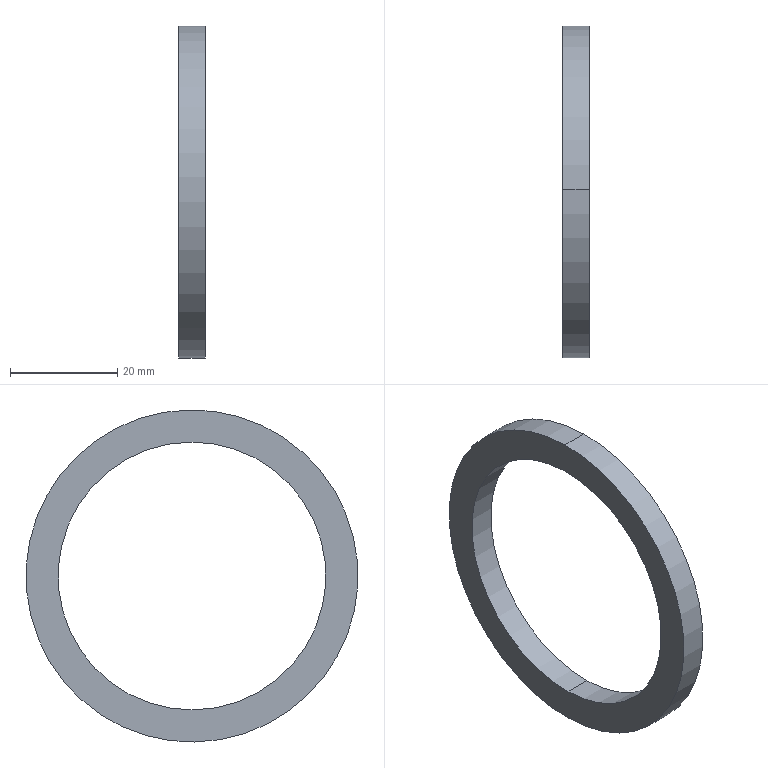Component | SolidWorks | Washer-1 | 1 solid | 6 faces | box 5 x 62 x 62 mm | volume 5278 mm3 | cylinder 4 | plane 2 | commonest cylinder face diameters 50 x2 62 x2
build123d program:
from build123d import *

# Parameters (mm, degrees)
SKETCH2_R           = 31
SKETCH2_R_2         = 25
BOSS_EXTRUDE1_DEPTH = 5


with BuildPart() as part:
    # Sketch2 → Boss-Extrude1 (new body)
    with BuildSketch(Plane.XY):
        with Locations((15, 150)):
            Circle(SKETCH2_R)
        with Locations((15, 150)):
            Circle(SKETCH2_R_2, mode=Mode.SUBTRACT)
    extrude(amount=BOSS_EXTRUDE1_DEPTH)


solid = part.part

# Placed as in the assembly
solid = solid.moved(Location((112.554, 0, 0), (0, 90, 0)))
STEP:
#1=CARTESIAN_POINT('',(4.628,5.92,0.3936));
#2=VERTEX_POINT('',#1);
#3=CARTESIAN_POINT('',(4.628,5.891,-1.575));
#4=VERTEX_POINT('',#3);
#5=CARTESIAN_POINT('',(4.628,5.906,-0.5906));
#6=DIRECTION('',(1.,0.,0.));
#7=DIRECTION('',(0.,-0.01499,-0.9999));
#8=AXIS2_PLACEMENT_3D('',#5,#6,#7);
#9=CIRCLE('',#8,0.9843);
#10=EDGE_CURVE('',#2,#4,#9,.T.);
#11=ORIENTED_EDGE('',*,*,#10,.T.);
#12=CARTESIAN_POINT('',(4.431,5.891,-1.575));
#13=VERTEX_POINT('',#12);
#14=CARTESIAN_POINT('',(4.628,5.891,-1.575));
#15=DIRECTION('',(-1.,-0.,-0.));
#16=VECTOR('',#15,39.37);
#17=LINE('',#14,#16);
#18=EDGE_CURVE('',#4,#13,#17,.T.);
#19=ORIENTED_EDGE('',*,*,#18,.T.);
#20=CARTESIAN_POINT('',(4.431,5.92,0.3936));
#21=VERTEX_POINT('',#20);
#22=CARTESIAN_POINT('',(4.431,5.906,-0.5906));
#23=DIRECTION('',(1.,0.,0.));
#24=DIRECTION('',(0.,-0.01499,-0.9999));
#25=AXIS2_PLACEMENT_3D('',#22,#23,#24);
#26=CIRCLE('',#25,0.9843);
#27=EDGE_CURVE('',#21,#13,#26,.T.);
#28=ORIENTED_EDGE('',*,*,#27,.F.);
#29=CARTESIAN_POINT('',(4.628,5.92,0.3936));
#30=DIRECTION('',(-1.,-0.,-0.));
#31=VECTOR('',#30,39.37);
#32=LINE('',#29,#31);
#33=EDGE_CURVE('',#2,#21,#32,.T.);
#34=ORIENTED_EDGE('',*,*,#33,.F.);
#35=EDGE_LOOP('',(#11,#19,#28,#34));
#36=FACE_OUTER_BOUND('',#35,.T.);
#37=CARTESIAN_POINT('',(4.628,5.906,-0.5906));
#38=DIRECTION('',(-1.,-0.,-0.));
#39=DIRECTION('',(0.,0.01499,0.9999));
#40=AXIS2_PLACEMENT_3D('',#37,#38,#39);
#41=CYLINDRICAL_SURFACE('',#40,0.9843);
#42=ADVANCED_FACE('',(#36),#41,.F.);
#43=CARTESIAN_POINT('',(4.628,5.887,-1.811));
#44=VERTEX_POINT('',#43);
#45=CARTESIAN_POINT('',(4.628,5.924,0.6298));
#46=VERTEX_POINT('',#45);
#47=CARTESIAN_POINT('',(4.628,5.906,-0.5906));
#48=DIRECTION('',(1.,0.,0.));
#49=DIRECTION('',(0.,-0.01499,-0.9999));
#50=AXIS2_PLACEMENT_3D('',#47,#48,#49);
#51=CIRCLE('',#50,1.22);
#52=EDGE_CURVE('',#44,#46,#51,.T.);
#53=ORIENTED_EDGE('',*,*,#52,.F.);
#54=CARTESIAN_POINT('',(4.431,5.887,-1.811));
#55=VERTEX_POINT('',#54);
#56=CARTESIAN_POINT('',(4.628,5.887,-1.811));
#57=DIRECTION('',(-1.,-0.,-0.));
#58=VECTOR('',#57,39.37);
#59=LINE('',#56,#58);
#60=EDGE_CURVE('',#44,#55,#59,.T.);
#61=ORIENTED_EDGE('',*,*,#60,.T.);
#62=CARTESIAN_POINT('',(4.431,5.924,0.6298));
#63=VERTEX_POINT('',#62);
#64=CARTESIAN_POINT('',(4.431,5.906,-0.5906));
#65=DIRECTION('',(1.,0.,0.));
#66=DIRECTION('',(0.,-0.01499,-0.9999));
#67=AXIS2_PLACEMENT_3D('',#64,#65,#66);
#68=CIRCLE('',#67,1.22);
#69=EDGE_CURVE('',#55,#63,#68,.T.);
#70=ORIENTED_EDGE('',*,*,#69,.T.);
#71=CARTESIAN_POINT('',(4.628,5.924,0.6298));
#72=DIRECTION('',(-1.,-0.,-0.));
#73=VECTOR('',#72,39.37);
#74=LINE('',#71,#73);
#75=EDGE_CURVE('',#46,#63,#74,.T.);
#76=ORIENTED_EDGE('',*,*,#75,.F.);
#77=EDGE_LOOP('',(#53,#61,#70,#76));
#78=FACE_OUTER_BOUND('',#77,.T.);
#79=CARTESIAN_POINT('',(4.628,5.906,-0.5906));
#80=DIRECTION('',(-1.,-0.,-0.));
#81=DIRECTION('',(0.,0.01499,0.9999));
#82=AXIS2_PLACEMENT_3D('',#79,#80,#81);
#83=CYLINDRICAL_SURFACE('',#82,1.22);
#84=ADVANCED_FACE('',(#78),#83,.T.);
#85=CARTESIAN_POINT('',(4.628,5.906,-0.5906));
#86=DIRECTION('',(1.,0.,0.));
#87=DIRECTION('',(0.,-0.01499,-0.9999));
#88=AXIS2_PLACEMENT_3D('',#85,#86,#87);
#89=CIRCLE('',#88,1.22);
#90=EDGE_CURVE('',#46,#44,#89,.T.);
#91=ORIENTED_EDGE('',*,*,#90,.T.);
#92=ORIENTED_EDGE('',*,*,#52,.T.);
#93=EDGE_LOOP('',(#91,#92));
#94=FACE_OUTER_BOUND('',#93,.T.);
#95=ORIENTED_EDGE('',*,*,#10,.F.);
#96=CARTESIAN_POINT('',(4.628,5.906,-0.5906));
#97=DIRECTION('',(1.,0.,0.));
#98=DIRECTION('',(0.,-0.01499,-0.9999));
#99=AXIS2_PLACEMENT_3D('',#96,#97,#98);
#100=CIRCLE('',#99,0.9843);
#101=EDGE_CURVE('',#4,#2,#100,.T.);
#102=ORIENTED_EDGE('',*,*,#101,.F.);
#103=EDGE_LOOP('',(#95,#102));
#104=FACE_BOUND('',#103,.T.);
#105=CARTESIAN_POINT('',(4.628,5.906,-0.5906));
#106=DIRECTION('',(1.,0.,0.));
#107=DIRECTION('',(0.,-0.01499,-0.9999));
#108=AXIS2_PLACEMENT_3D('',#105,#106,#107);
#109=PLANE('',#108);
#110=ADVANCED_FACE('',(#94,#104),#109,.T.);
#111=CARTESIAN_POINT('',(4.431,5.906,-0.5906));
#112=DIRECTION('',(1.,0.,0.));
#113=DIRECTION('',(0.,-0.01499,-0.9999));
#114=AXIS2_PLACEMENT_3D('',#111,#112,#113);
#115=CIRCLE('',#114,1.22);
#116=EDGE_CURVE('',#63,#55,#115,.T.);
#117=ORIENTED_EDGE('',*,*,#116,.F.);
#118=ORIENTED_EDGE('',*,*,#69,.F.);
#119=EDGE_LOOP('',(#117,#118));
#120=FACE_OUTER_BOUND('',#119,.T.);
#121=ORIENTED_EDGE('',*,*,#27,.T.);
#122=CARTESIAN_POINT('',(4.431,5.906,-0.5906));
#123=DIRECTION('',(1.,0.,0.));
#124=DIRECTION('',(0.,-0.01499,-0.9999));
#125=AXIS2_PLACEMENT_3D('',#122,#123,#124);
#126=CIRCLE('',#125,0.9843);
#127=EDGE_CURVE('',#13,#21,#126,.T.);
#128=ORIENTED_EDGE('',*,*,#127,.T.);
#129=EDGE_LOOP('',(#121,#128));
#130=FACE_BOUND('',#129,.T.);
#131=CARTESIAN_POINT('',(4.431,5.906,-0.5906));
#132=DIRECTION('',(1.,0.,0.));
#133=DIRECTION('',(0.,-0.01499,-0.9999));
#134=AXIS2_PLACEMENT_3D('',#131,#132,#133);
#135=PLANE('',#134);
#136=ADVANCED_FACE('',(#120,#130),#135,.F.);
#137=ORIENTED_EDGE('',*,*,#60,.F.);
#138=ORIENTED_EDGE('',*,*,#90,.F.);
#139=ORIENTED_EDGE('',*,*,#75,.T.);
#140=ORIENTED_EDGE('',*,*,#116,.T.);
#141=EDGE_LOOP('',(#137,#138,#139,#140));
#142=FACE_OUTER_BOUND('',#141,.T.);
#143=CARTESIAN_POINT('',(4.628,5.906,-0.5906));
#144=DIRECTION('',(-1.,-0.,-0.));
#145=DIRECTION('',(0.,0.01499,0.9999));
#146=AXIS2_PLACEMENT_3D('',#143,#144,#145);
#147=CYLINDRICAL_SURFACE('',#146,1.22);
#148=ADVANCED_FACE('',(#142),#147,.T.);
#149=ORIENTED_EDGE('',*,*,#18,.F.);
#150=ORIENTED_EDGE('',*,*,#101,.T.);
#151=ORIENTED_EDGE('',*,*,#33,.T.);
#152=ORIENTED_EDGE('',*,*,#127,.F.);
#153=EDGE_LOOP('',(#149,#150,#151,#152));
#154=FACE_OUTER_BOUND('',#153,.T.);
#155=CARTESIAN_POINT('',(4.628,5.906,-0.5906));
#156=DIRECTION('',(-1.,-0.,-0.));
#157=DIRECTION('',(0.,0.01499,0.9999));
#158=AXIS2_PLACEMENT_3D('',#155,#156,#157);
#159=CYLINDRICAL_SURFACE('',#158,0.9843);
#160=ADVANCED_FACE('',(#154),#159,.F.);
#161=CLOSED_SHELL('',(#42,#84,#110,#136,#148,#160));
#162=MANIFOLD_SOLID_BREP('',#161);
#163=CARTESIAN_POINT('',(0.,0.,0.));
#164=DIRECTION('',(0.,0.,1.));
#165=DIRECTION('',(1.,0.,0.));
#166=AXIS2_PLACEMENT_3D('',#163,#164,#165);
#167=(LENGTH_UNIT()NAMED_UNIT(*)SI_UNIT($,.METRE.));
#168=LENGTH_MEASURE_WITH_UNIT(LENGTH_MEASURE(0.0254),#167);
#169=DIMENSIONAL_EXPONENTS(1.,0.,0.,0.,0.,0.,0.);
#170=(CONVERSION_BASED_UNIT('',#168)LENGTH_UNIT()NAMED_UNIT(#169));
#171=UNCERTAINTY_MEASURE_WITH_UNIT(LENGTH_MEASURE(0.00001),#170,'','');
#172=(NAMED_UNIT(*)PLANE_ANGLE_UNIT()SI_UNIT($,.RADIAN.));
#173=(NAMED_UNIT(*)SI_UNIT($,.STERADIAN.)SOLID_ANGLE_UNIT());
#174=(GEOMETRIC_REPRESENTATION_CONTEXT(3)GLOBAL_UNCERTAINTY_ASSIGNED_CONTEXT((#171))GLOBAL_UNIT_ASSIGNED_CONTEXT((#170,#172,#173))REPRESENTATION_CONTEXT('',''));
#175=ADVANCED_BREP_SHAPE_REPRESENTATION('',(#162,#166),#174);
#176=COLOUR_RGB('',0.7922,0.8196,0.9333);
#177=FILL_AREA_STYLE_COLOUR('',#176);
#178=FILL_AREA_STYLE('',(#177));
#179=SURFACE_STYLE_FILL_AREA(#178);
#180=SURFACE_SIDE_STYLE('',(#179));
#181=SURFACE_STYLE_USAGE(.BOTH.,#180);
#182=PRESENTATION_STYLE_ASSIGNMENT((#181));
#183=STYLED_ITEM('',(#182),#162);
#184=(LENGTH_UNIT()NAMED_UNIT(*)SI_UNIT($,.METRE.));
#185=LENGTH_MEASURE_WITH_UNIT(LENGTH_MEASURE(0.0254),#184);
#186=DIMENSIONAL_EXPONENTS(1.,0.,0.,0.,0.,0.,0.);
#187=(CONVERSION_BASED_UNIT('',#185)LENGTH_UNIT()NAMED_UNIT(#186));
#188=UNCERTAINTY_MEASURE_WITH_UNIT(LENGTH_MEASURE(0.00001),#187,'','');
#189=(NAMED_UNIT(*)PLANE_ANGLE_UNIT()SI_UNIT($,.RADIAN.));
#190=(NAMED_UNIT(*)SI_UNIT($,.STERADIAN.)SOLID_ANGLE_UNIT());
#191=(GEOMETRIC_REPRESENTATION_CONTEXT(3)GLOBAL_UNCERTAINTY_ASSIGNED_CONTEXT((#188))GLOBAL_UNIT_ASSIGNED_CONTEXT((#187,#189,#190))REPRESENTATION_CONTEXT('',''));
#192=MECHANICAL_DESIGN_GEOMETRIC_PRESENTATION_REPRESENTATION('',(#183),#191);
#193=PRESENTATION_LAYER_ASSIGNMENT('','',(#183));